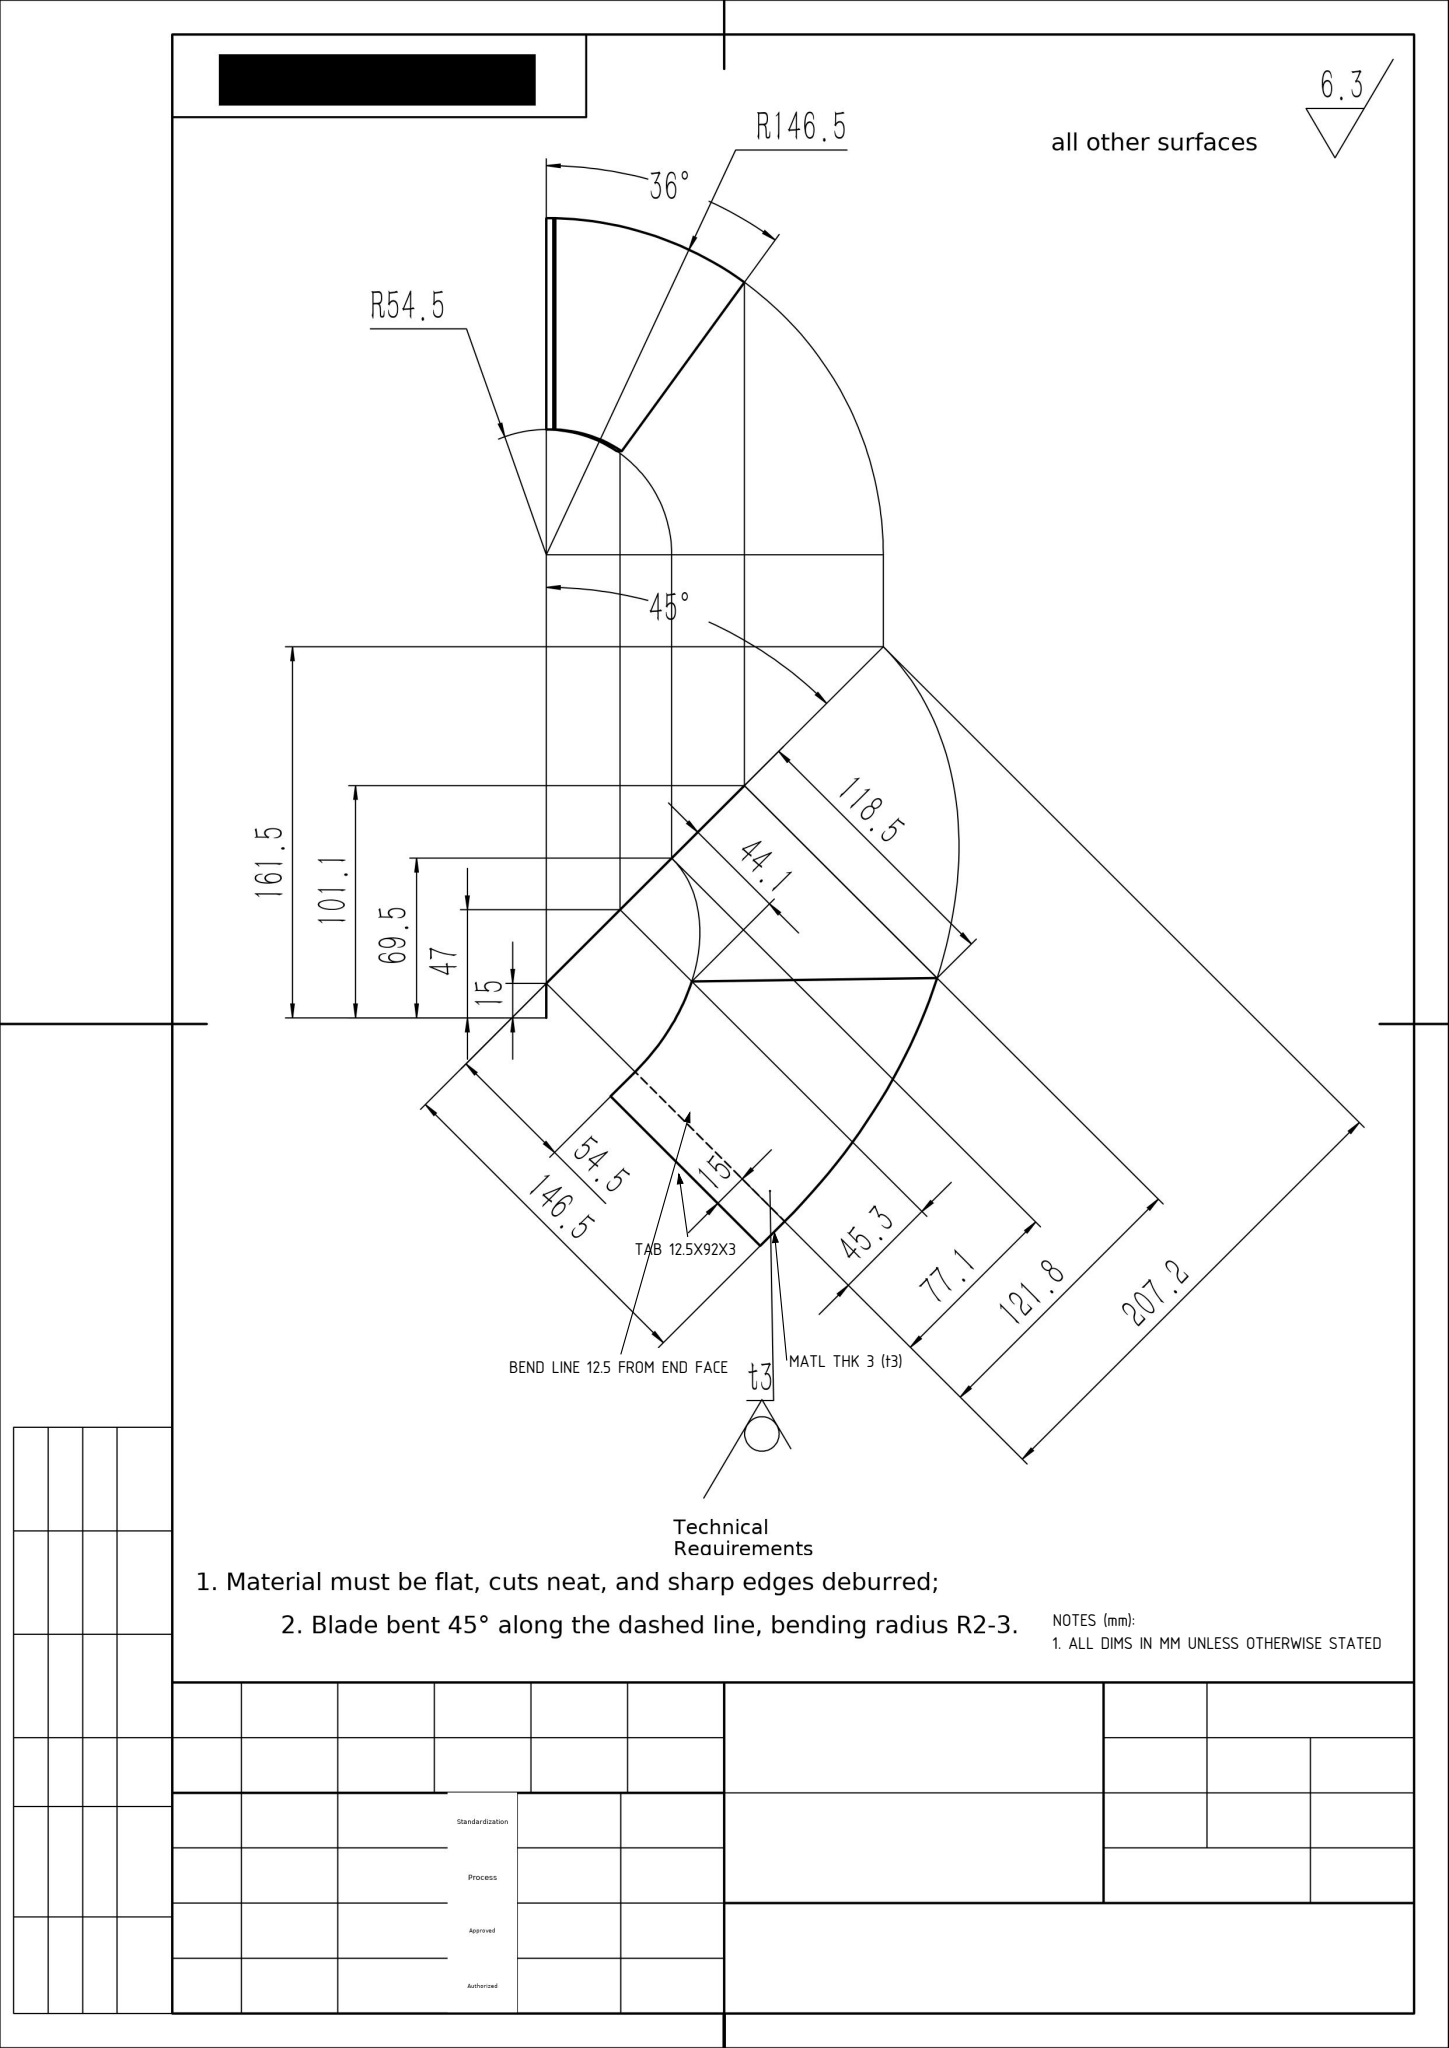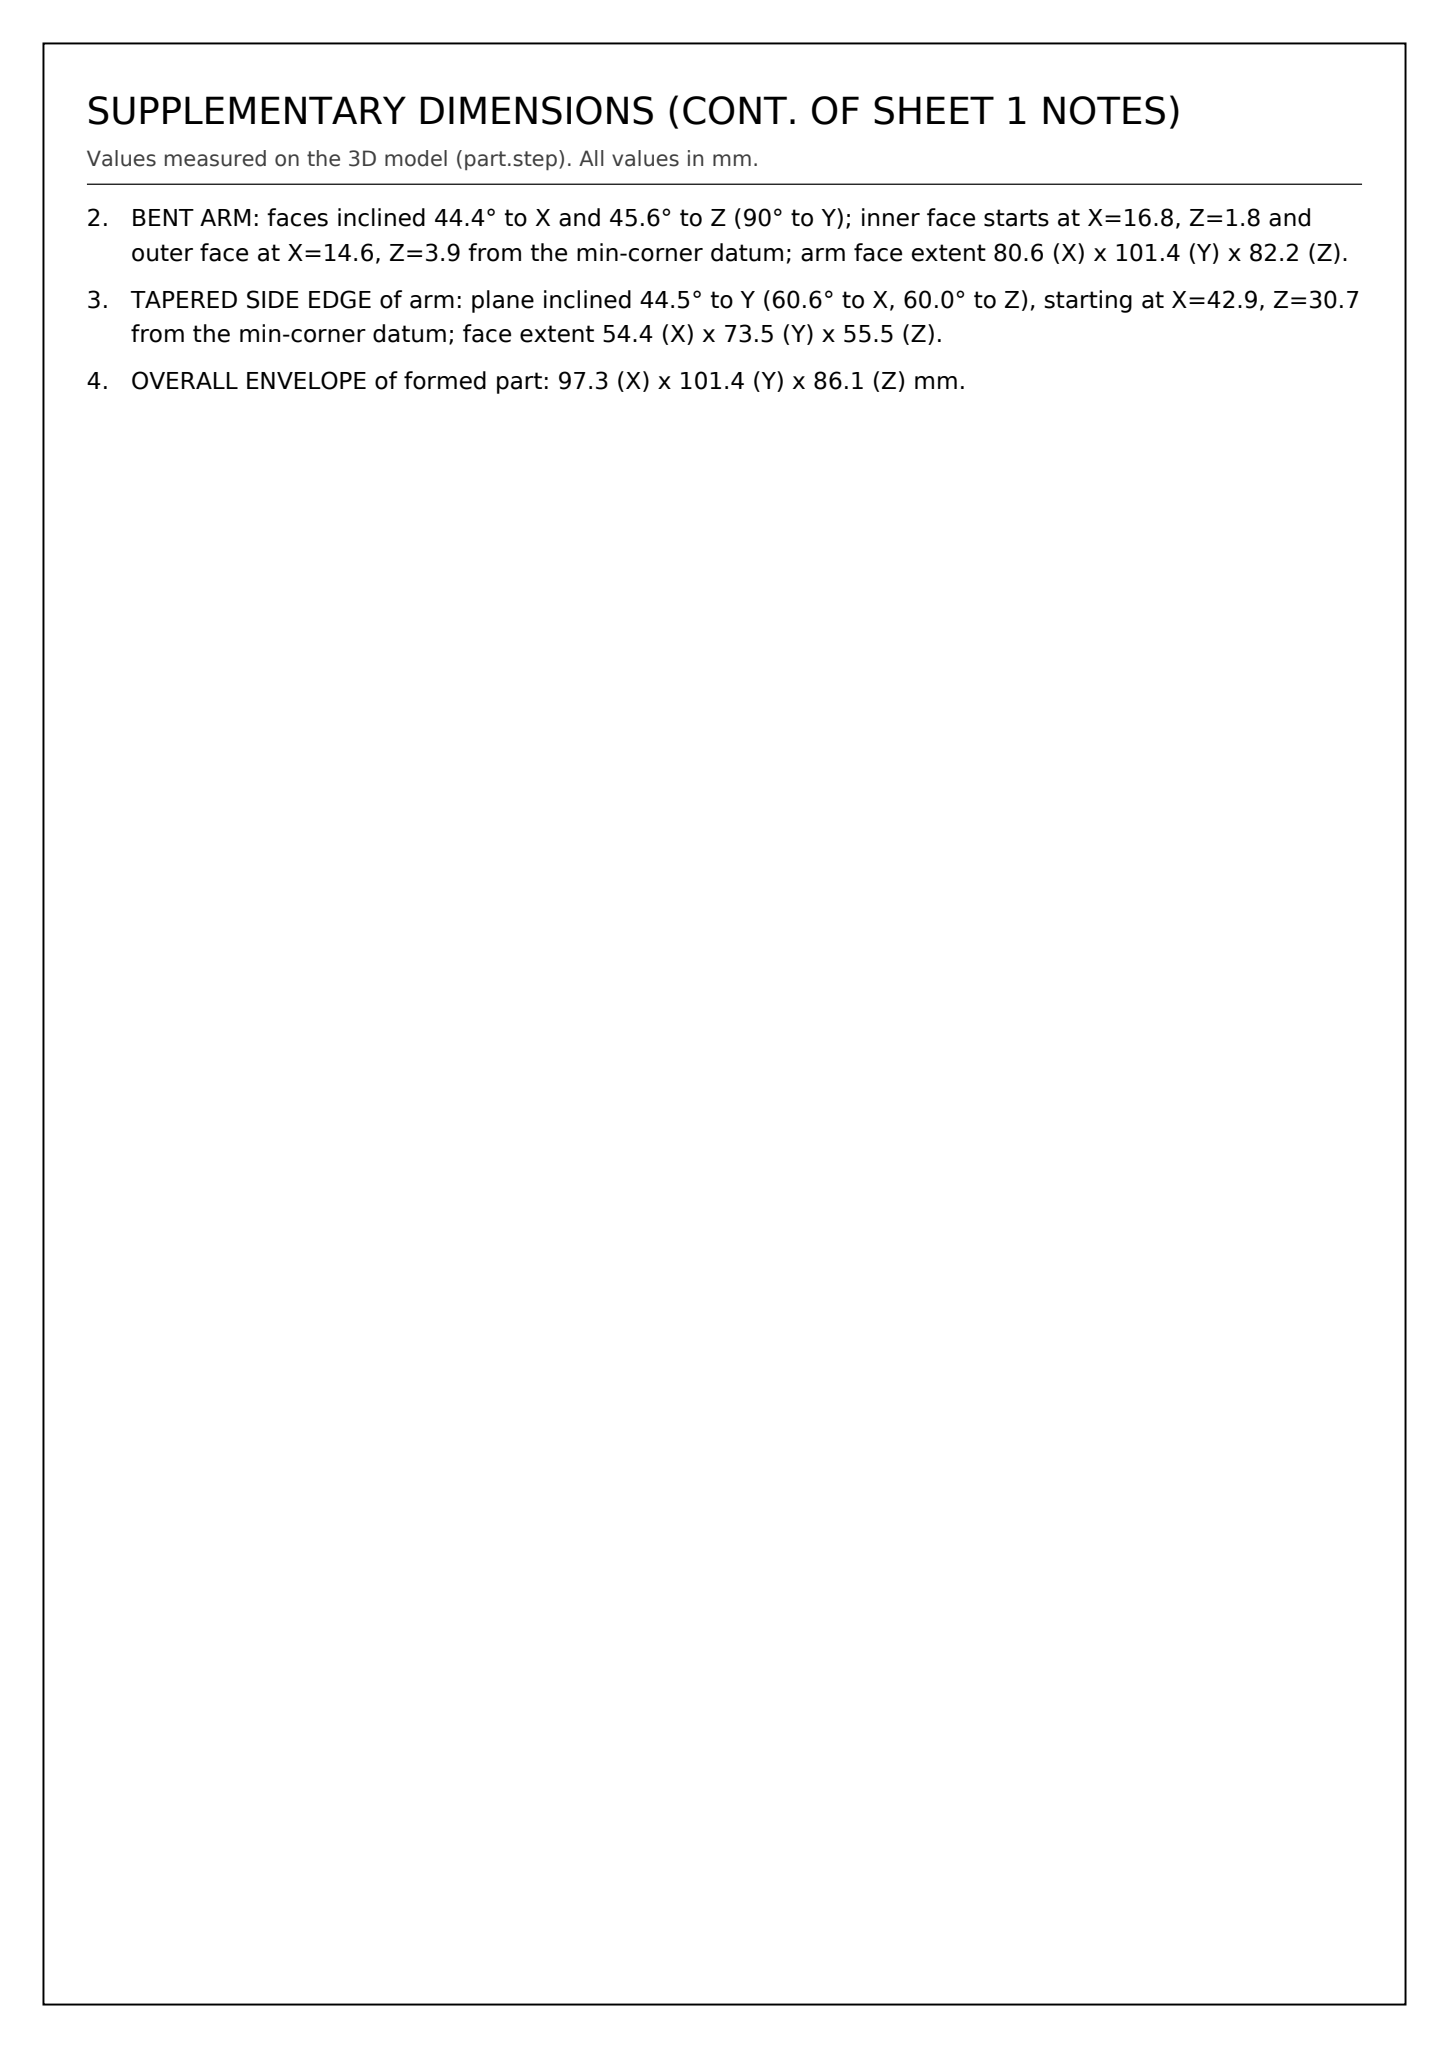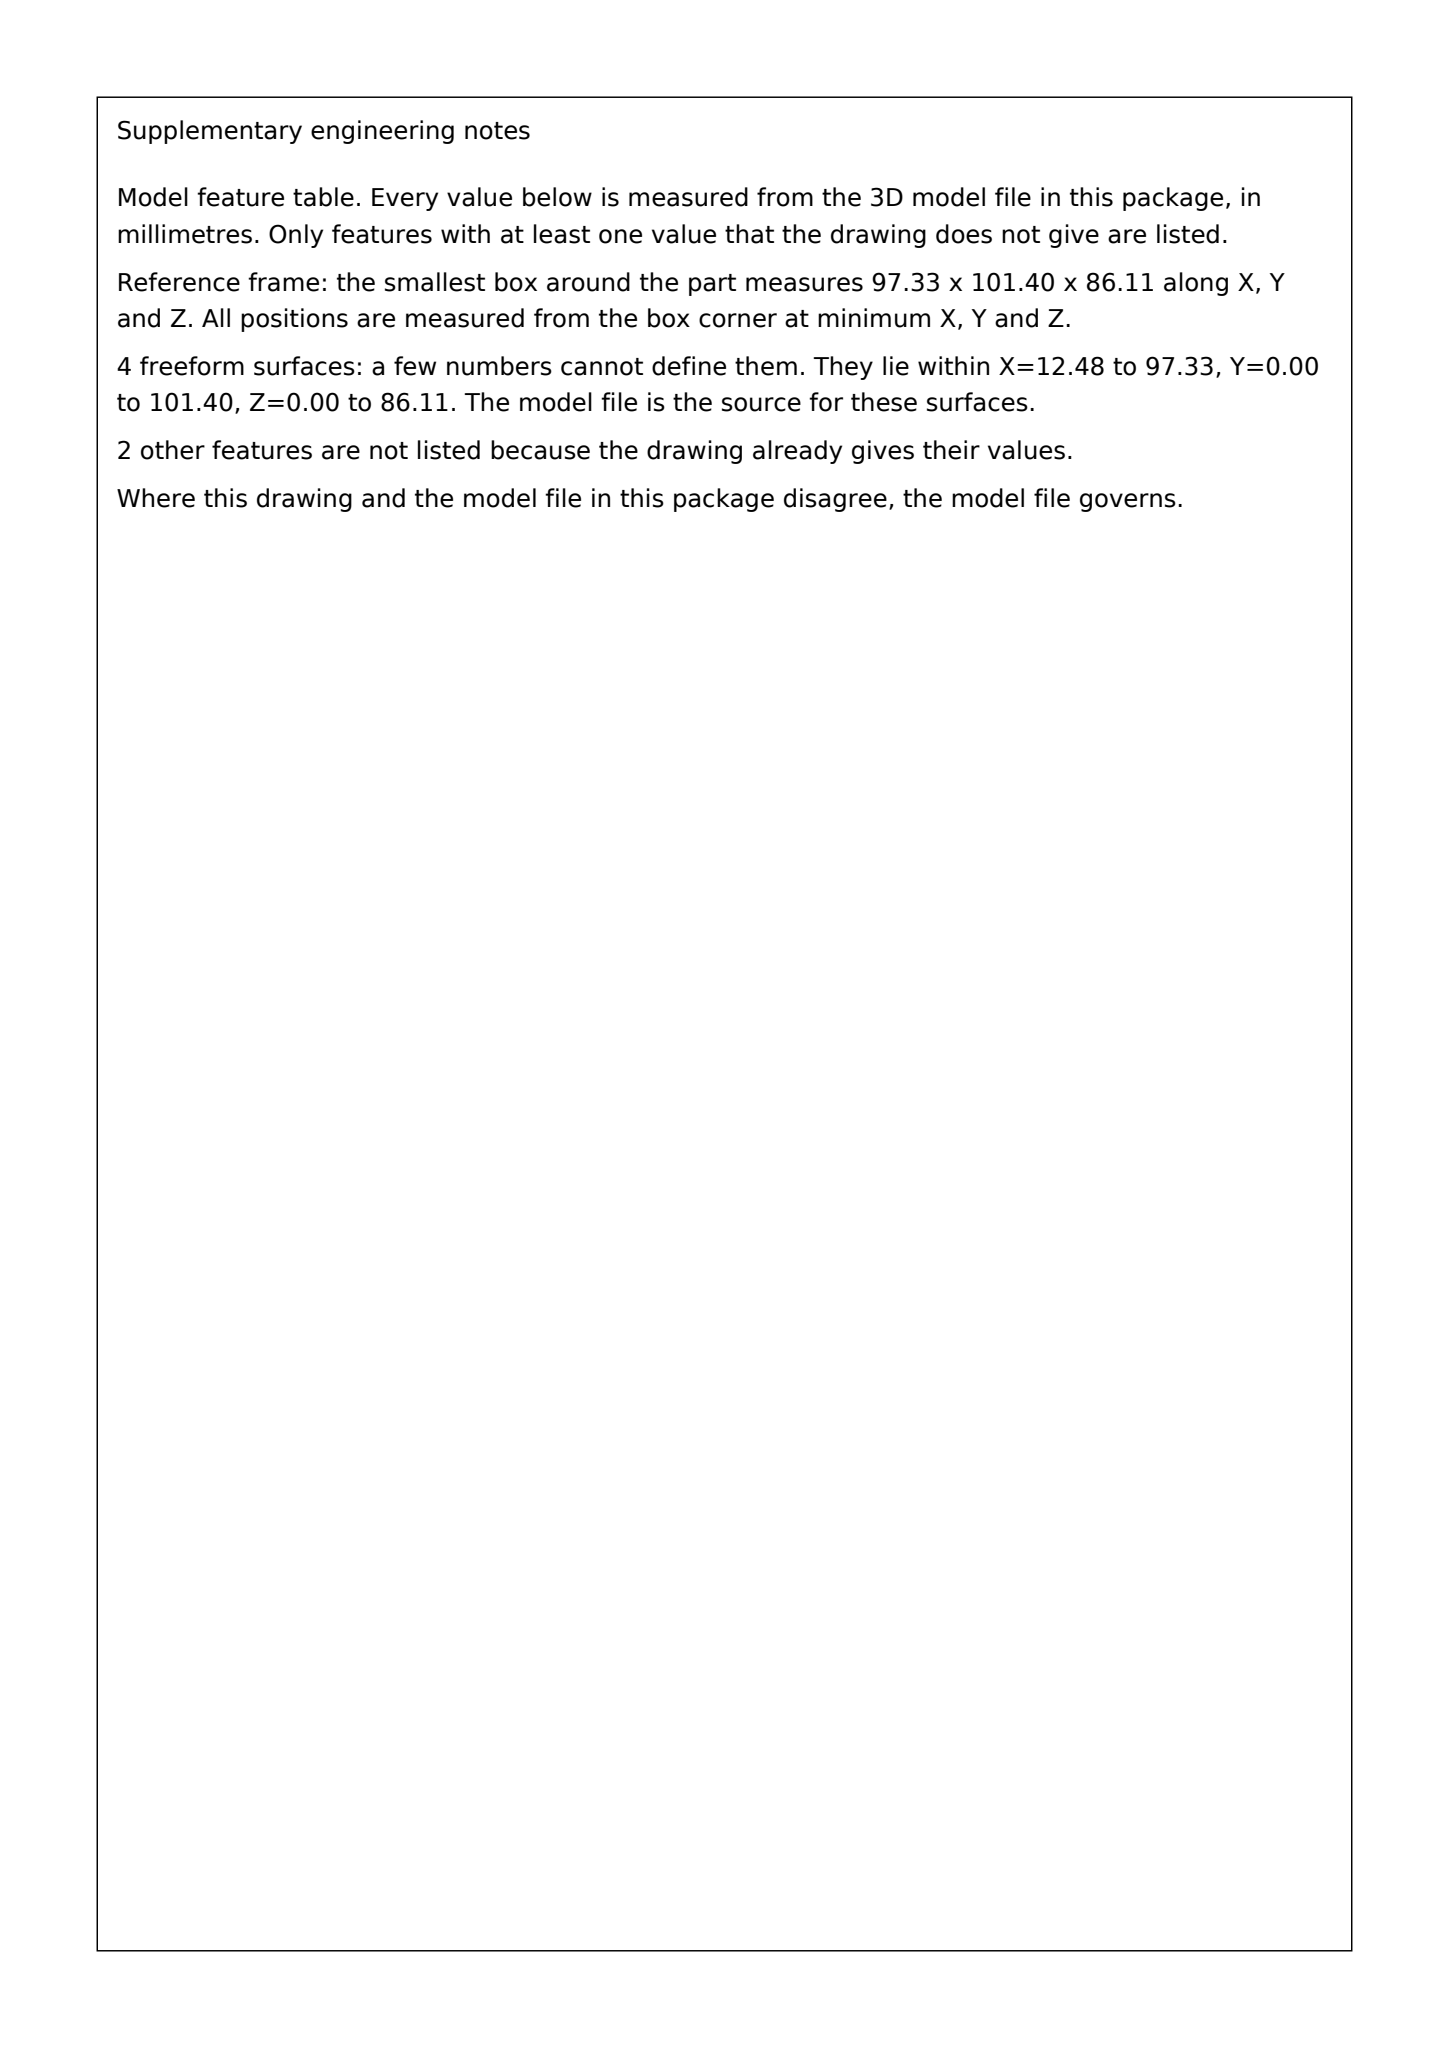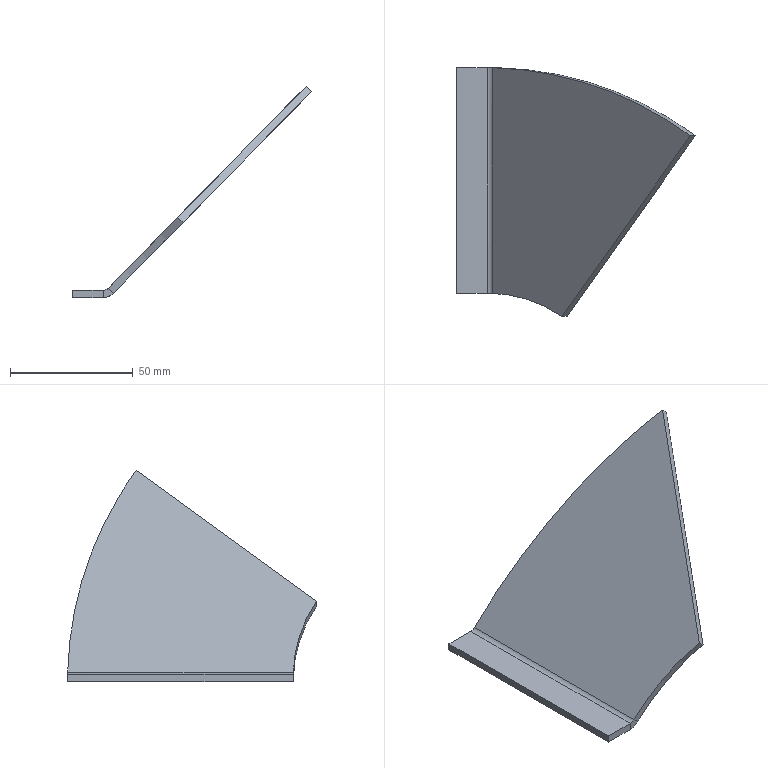Part | SolidWorks | mm | 1 solid | 14 faces | box 97.33 x 101.4 x 86.11 mm | volume 27238 mm3 | plane 8 | spline 4 | cylinder 2 | commonest cylinder face diameters 12 x1 6 x1
Drawing notes:
ALL DIMS IN MM UNLESS OTHERWISE STATED | from the solid: STEP model in mm: plate thk 3.00 (z 0.03 to 3.03) = drawing t3; bbox 97.331 x 101.401 x 86.141 consistent with 146.5/54.5 arc dims in mm
BENT ARM: faces inclined 44.4° to X and 45.6° to Z (90° to Y); inner face starts at X=16.8, Z=1.8 and outer face at X=14.6, Z=3.9 from the min-corner datum; arm face extent 80.6 (X) x 101.4 (Y) x 82.2 (Z). | from the solid: inclined_planes angle_to_xyz_axes [44.4,90.0,45.6], bbox_from [14.6,0.0,3.9] and [16.8,0.0,1.8], size [80.6,101.4,82.2]
TAPERED SIDE EDGE of arm: plane inclined 44.5° to Y (60.6° to X, 60.0° to Z), starting at X=42.9, Z=30.7 from the min-corner datum; face extent 54.4 (X) x 73.5 (Y) x 55.5 (Z). | from the solid: inclined_planes angle_to_xyz_axes [60.6,44.5,60.0], bbox_from [42.9,0.0,30.7], size [54.4,73.5,55.5]
OVERALL ENVELOPE of formed part: 97.3 (X) x 101.4 (Y) x 86.1 (Z) mm. | from the solid: bbox_xyz [97.331,101.401,86.141]
FLAT TAB 12.5X92X3: START 9.4 FROM END OF 101.4 EDGE | from the solid: Planes z=0/3 extent x[0,12.5] y[9.4,101.4]; bbox y=101.401
MATL THK 3 (t3) - RELOCATE CALLOUT CLEAR OF EXT LINES | from the solid: Tab faces z=0 and z=3, thickness 3
BEND LINE 12.5 FROM END FACE (DELETE 15) | from the solid: Tab x extent 0 to 12.5; arc axes at x=12.5
STEP:
#1=CARTESIAN_POINT('',(-147.378,146.448,3.9));
#2=VERTEX_POINT('',#1);
#3=CARTESIAN_POINT('',(-66.812,118.521,86.111));
#4=VERTEX_POINT('',#3);
#5=CARTESIAN_POINT('',(-147.378,146.448,3.9));
#6=CARTESIAN_POINT('',(-118.151,145.654,33.724));
#7=CARTESIAN_POINT('',(-90.466,136.057,61.974));
#8=CARTESIAN_POINT('',(-66.812,118.521,86.111));
#9=(BOUNDED_CURVE()B_SPLINE_CURVE(3,(#5,#6,#7,#8),.UNSPECIFIED.,.F.,.F.)B_SPLINE_CURVE_WITH_KNOTS((4,4),(4.739,5.341),.UNSPECIFIED.)CURVE()GEOMETRIC_REPRESENTATION_ITEM()RATIONAL_B_SPLINE_CURVE((1.,0.9701,0.9701,1.))REPRESENTATION_ITEM(''));
#10=EDGE_CURVE('',#2,#4,#9,.T.);
#11=ORIENTED_EDGE('',*,*,#10,.F.);
#12=CARTESIAN_POINT('',(-147.378,54.47,3.9));
#13=VERTEX_POINT('',#12);
#14=CARTESIAN_POINT('',(-147.378,147.,3.9));
#15=DIRECTION('',(0.,-1.,0.));
#16=VECTOR('',#15,1000.);
#17=LINE('',#14,#16);
#18=EDGE_CURVE('',#2,#13,#17,.T.);
#19=ORIENTED_EDGE('',*,*,#18,.T.);
#20=CARTESIAN_POINT('',(-119.111,45.069,32.744));
#21=VERTEX_POINT('',#20);
#22=CARTESIAN_POINT('',(-119.111,45.069,32.744));
#23=CARTESIAN_POINT('',(-127.528,50.908,24.155));
#24=CARTESIAN_POINT('',(-137.205,54.127,14.281));
#25=CARTESIAN_POINT('',(-147.378,54.47,3.9));
#26=(BOUNDED_CURVE()B_SPLINE_CURVE(3,(#22,#23,#24,#25),.UNSPECIFIED.,.F.,.F.)B_SPLINE_CURVE_WITH_KNOTS((4,4),(0.9737,1.538),.UNSPECIFIED.)CURVE()GEOMETRIC_REPRESENTATION_ITEM()RATIONAL_B_SPLINE_CURVE((1.,0.9737,0.9737,1.))REPRESENTATION_ITEM(''));
#27=EDGE_CURVE('',#21,#13,#26,.T.);
#28=ORIENTED_EDGE('',*,*,#27,.F.);
#29=CARTESIAN_POINT('',(-98.717,73.712,53.555));
#30=DIRECTION('',(-0.4991,-0.701,-0.5093));
#31=VECTOR('',#30,1000.);
#32=LINE('',#29,#31);
#33=EDGE_CURVE('',#4,#21,#32,.T.);
#34=ORIENTED_EDGE('',*,*,#33,.F.);
#35=EDGE_LOOP('',(#11,#19,#28,#34));
#36=FACE_OUTER_BOUND('',#35,.T.);
#37=CARTESIAN_POINT('',(-149.143,147.,2.1));
#38=DIRECTION('',(0.7142,0.,-0.6999));
#39=DIRECTION('',(-0.6999,0.,-0.7142));
#40=AXIS2_PLACEMENT_3D('',#37,#38,#39);
#41=PLANE('',#40);
#42=ADVANCED_FACE('',(#36),#41,.F.);
#43=CARTESIAN_POINT('',(-145.236,146.448,1.8));
#44=VERTEX_POINT('',#43);
#45=CARTESIAN_POINT('',(-145.236,54.47,1.8));
#46=VERTEX_POINT('',#45);
#47=CARTESIAN_POINT('',(-145.236,147.,1.8));
#48=DIRECTION('',(0.,-1.,0.));
#49=VECTOR('',#48,1000.);
#50=LINE('',#47,#49);
#51=EDGE_CURVE('',#44,#46,#50,.T.);
#52=ORIENTED_EDGE('',*,*,#51,.F.);
#53=CARTESIAN_POINT('',(-64.669,118.521,84.011));
#54=VERTEX_POINT('',#53);
#55=CARTESIAN_POINT('',(-145.236,146.448,1.8));
#56=CARTESIAN_POINT('',(-116.008,145.654,31.625));
#57=CARTESIAN_POINT('',(-88.324,136.057,59.874));
#58=CARTESIAN_POINT('',(-64.669,118.521,84.011));
#59=(BOUNDED_CURVE()B_SPLINE_CURVE(3,(#55,#56,#57,#58),.UNSPECIFIED.,.F.,.T.)B_SPLINE_CURVE_WITH_KNOTS((4,4),(4.739,5.341),.UNSPECIFIED.)CURVE()GEOMETRIC_REPRESENTATION_ITEM()RATIONAL_B_SPLINE_CURVE((1.,0.9701,0.9701,1.))REPRESENTATION_ITEM(''));
#60=EDGE_CURVE('',#44,#54,#59,.T.);
#61=ORIENTED_EDGE('',*,*,#60,.T.);
#62=CARTESIAN_POINT('',(-116.968,45.069,30.644));
#63=VERTEX_POINT('',#62);
#64=CARTESIAN_POINT('',(-96.574,73.712,51.455));
#65=DIRECTION('',(-0.4991,-0.701,-0.5093));
#66=VECTOR('',#65,1000.);
#67=LINE('',#64,#66);
#68=EDGE_CURVE('',#54,#63,#67,.T.);
#69=ORIENTED_EDGE('',*,*,#68,.T.);
#70=CARTESIAN_POINT('',(-116.968,45.069,30.644));
#71=CARTESIAN_POINT('',(-125.385,50.908,22.056));
#72=CARTESIAN_POINT('',(-135.063,54.127,12.181));
#73=CARTESIAN_POINT('',(-145.236,54.47,1.8));
#74=(BOUNDED_CURVE()B_SPLINE_CURVE(3,(#70,#71,#72,#73),.UNSPECIFIED.,.F.,.F.)B_SPLINE_CURVE_WITH_KNOTS((4,4),(0.9737,1.538),.UNSPECIFIED.)CURVE()GEOMETRIC_REPRESENTATION_ITEM()RATIONAL_B_SPLINE_CURVE((1.,0.9737,0.9737,1.))REPRESENTATION_ITEM(''));
#75=EDGE_CURVE('',#63,#46,#74,.T.);
#76=ORIENTED_EDGE('',*,*,#75,.T.);
#77=EDGE_LOOP('',(#52,#61,#69,#76));
#78=FACE_OUTER_BOUND('',#77,.T.);
#79=CARTESIAN_POINT('',(-147.,147.,0.));
#80=DIRECTION('',(0.7142,0.,-0.6999));
#81=DIRECTION('',(-0.6999,0.,-0.7142));
#82=AXIS2_PLACEMENT_3D('',#79,#80,#81);
#83=PLANE('',#82);
#84=ADVANCED_FACE('',(#78),#83,.T.);
#85=CARTESIAN_POINT('',(-149.521,146.469,0.));
#86=VERTEX_POINT('',#85);
#87=CARTESIAN_POINT('',(-149.521,54.5,0.));
#88=VERTEX_POINT('',#87);
#89=CARTESIAN_POINT('',(-149.521,147.,0.));
#90=DIRECTION('',(0.,-1.,0.));
#91=VECTOR('',#90,1000.);
#92=LINE('',#89,#91);
#93=EDGE_CURVE('',#86,#88,#92,.T.);
#94=ORIENTED_EDGE('',*,*,#93,.F.);
#95=CARTESIAN_POINT('',(-149.521,146.469,0.));
#96=CARTESIAN_POINT('',(-149.12,146.469,0.));
#97=CARTESIAN_POINT('',(-148.726,146.469,0.03981));
#98=CARTESIAN_POINT('',(-148.144,146.468,0.1568));
#99=CARTESIAN_POINT('',(-147.952,146.467,0.2054));
#100=CARTESIAN_POINT('',(-147.57,146.466,0.3224));
#101=CARTESIAN_POINT('',(-147.381,146.465,0.3909));
#102=CARTESIAN_POINT('',(-146.831,146.463,0.6219));
#103=CARTESIAN_POINT('',(-146.484,146.46,0.8103));
#104=CARTESIAN_POINT('',(-145.826,146.455,1.256));
#105=CARTESIAN_POINT('',(-145.516,146.452,1.514));
#106=CARTESIAN_POINT('',(-145.236,146.448,1.8));
#107=B_SPLINE_CURVE_WITH_KNOTS('',3,(#95,#96,#97,#98,#99,#100,#101,#102,#103,#104,#105,#106),.UNSPECIFIED.,.F.,.F.,(4,2,2,2,2,4),(0.,0.001186,0.001779,0.002372,0.003558,0.004744),.UNSPECIFIED.);
#108=EDGE_CURVE('',#86,#44,#107,.T.);
#109=ORIENTED_EDGE('',*,*,#108,.T.);
#110=ORIENTED_EDGE('',*,*,#51,.T.);
#111=CARTESIAN_POINT('',(-145.236,54.47,1.8));
#112=CARTESIAN_POINT('',(-145.516,54.48,1.514));
#113=CARTESIAN_POINT('',(-145.821,54.486,1.26));
#114=CARTESIAN_POINT('',(-146.311,54.492,0.9268));
#115=CARTESIAN_POINT('',(-146.481,54.494,0.8235));
#116=CARTESIAN_POINT('',(-146.831,54.496,0.6331));
#117=CARTESIAN_POINT('',(-147.012,54.497,0.546));
#118=CARTESIAN_POINT('',(-147.562,54.499,0.3148));
#119=CARTESIAN_POINT('',(-147.94,54.5,0.1984));
#120=CARTESIAN_POINT('',(-148.718,54.5,0.04068));
#121=CARTESIAN_POINT('',(-149.12,54.5,0.));
#122=CARTESIAN_POINT('',(-149.521,54.5,0.));
#123=B_SPLINE_CURVE_WITH_KNOTS('',3,(#111,#112,#113,#114,#115,#116,#117,#118,#119,#120,#121,#122),.UNSPECIFIED.,.F.,.F.,(4,2,2,2,2,4),(0.,0.001186,0.001779,0.002372,0.003558,0.004745),.UNSPECIFIED.);
#124=EDGE_CURVE('',#46,#88,#123,.T.);
#125=ORIENTED_EDGE('',*,*,#124,.T.);
#126=EDGE_LOOP('',(#94,#109,#110,#125));
#127=FACE_OUTER_BOUND('',#126,.T.);
#128=CARTESIAN_POINT('',(-149.521,147.,6.));
#129=DIRECTION('',(0.,-1.,0.));
#130=DIRECTION('',(0.,0.,-1.));
#131=AXIS2_PLACEMENT_3D('',#128,#129,#130);
#132=CYLINDRICAL_SURFACE('',#131,6.);
#133=ADVANCED_FACE('',(#127),#132,.T.);
#134=CARTESIAN_POINT('',(-162.,146.469,0.));
#135=VERTEX_POINT('',#134);
#136=CARTESIAN_POINT('',(-162.,54.5,0.));
#137=VERTEX_POINT('',#136);
#138=CARTESIAN_POINT('',(-162.,147.,0.));
#139=DIRECTION('',(0.,-1.,0.));
#140=VECTOR('',#139,1000.);
#141=LINE('',#138,#140);
#142=EDGE_CURVE('',#135,#137,#141,.T.);
#143=ORIENTED_EDGE('',*,*,#142,.F.);
#144=CARTESIAN_POINT('',(-162.,146.469,0.));
#145=DIRECTION('',(1.,0.,0.));
#146=VECTOR('',#145,1000.);
#147=LINE('',#144,#146);
#148=EDGE_CURVE('',#135,#86,#147,.T.);
#149=ORIENTED_EDGE('',*,*,#148,.T.);
#150=ORIENTED_EDGE('',*,*,#93,.T.);
#151=CARTESIAN_POINT('',(-162.,54.5,0.));
#152=DIRECTION('',(1.,0.,0.));
#153=VECTOR('',#152,1000.);
#154=LINE('',#151,#153);
#155=EDGE_CURVE('',#137,#88,#154,.T.);
#156=ORIENTED_EDGE('',*,*,#155,.F.);
#157=EDGE_LOOP('',(#143,#149,#150,#156));
#158=FACE_OUTER_BOUND('',#157,.T.);
#159=CARTESIAN_POINT('',(-162.,147.,0.));
#160=DIRECTION('',(0.,0.,-1.));
#161=DIRECTION('',(-1.,0.,-0.));
#162=AXIS2_PLACEMENT_3D('',#159,#160,#161);
#163=PLANE('',#162);
#164=ADVANCED_FACE('',(#158),#163,.T.);
#165=CARTESIAN_POINT('',(-162.,146.469,3.));
#166=VERTEX_POINT('',#165);
#167=CARTESIAN_POINT('',(-162.,54.5,3.));
#168=VERTEX_POINT('',#167);
#169=CARTESIAN_POINT('',(-162.,147.,3.));
#170=DIRECTION('',(0.,-1.,0.));
#171=VECTOR('',#170,1000.);
#172=LINE('',#169,#171);
#173=EDGE_CURVE('',#166,#168,#172,.T.);
#174=ORIENTED_EDGE('',*,*,#173,.F.);
#175=CARTESIAN_POINT('',(-162.,146.469,3.));
#176=DIRECTION('',(0.,0.,-1.));
#177=VECTOR('',#176,1000.);
#178=LINE('',#175,#177);
#179=EDGE_CURVE('',#166,#135,#178,.T.);
#180=ORIENTED_EDGE('',*,*,#179,.T.);
#181=ORIENTED_EDGE('',*,*,#142,.T.);
#182=CARTESIAN_POINT('',(-162.,54.5,0.));
#183=DIRECTION('',(-0.,0.,1.));
#184=VECTOR('',#183,1000.);
#185=LINE('',#182,#184);
#186=EDGE_CURVE('',#137,#168,#185,.T.);
#187=ORIENTED_EDGE('',*,*,#186,.T.);
#188=EDGE_LOOP('',(#174,#180,#181,#187));
#189=FACE_OUTER_BOUND('',#188,.T.);
#190=CARTESIAN_POINT('',(-162.,147.,3.));
#191=DIRECTION('',(-1.,0.,0.));
#192=DIRECTION('',(0.,0.,1.));
#193=AXIS2_PLACEMENT_3D('',#190,#191,#192);
#194=PLANE('',#193);
#195=ADVANCED_FACE('',(#189),#194,.T.);
#196=CARTESIAN_POINT('',(-149.521,146.469,3.));
#197=VERTEX_POINT('',#196);
#198=CARTESIAN_POINT('',(-162.,146.469,3.));
#199=DIRECTION('',(1.,0.,0.));
#200=VECTOR('',#199,1000.);
#201=LINE('',#198,#200);
#202=EDGE_CURVE('',#166,#197,#201,.T.);
#203=ORIENTED_EDGE('',*,*,#202,.F.);
#204=ORIENTED_EDGE('',*,*,#173,.T.);
#205=CARTESIAN_POINT('',(-149.521,54.5,3.));
#206=VERTEX_POINT('',#205);
#207=CARTESIAN_POINT('',(-162.,54.5,3.));
#208=DIRECTION('',(1.,0.,0.));
#209=VECTOR('',#208,1000.);
#210=LINE('',#207,#209);
#211=EDGE_CURVE('',#168,#206,#210,.T.);
#212=ORIENTED_EDGE('',*,*,#211,.T.);
#213=CARTESIAN_POINT('',(-149.521,147.,3.));
#214=DIRECTION('',(0.,-1.,0.));
#215=VECTOR('',#214,1000.);
#216=LINE('',#213,#215);
#217=EDGE_CURVE('',#197,#206,#216,.T.);
#218=ORIENTED_EDGE('',*,*,#217,.F.);
#219=EDGE_LOOP('',(#203,#204,#212,#218));
#220=FACE_OUTER_BOUND('',#219,.T.);
#221=CARTESIAN_POINT('',(-162.,147.,3.));
#222=DIRECTION('',(0.,0.,-1.));
#223=DIRECTION('',(-1.,0.,-0.));
#224=AXIS2_PLACEMENT_3D('',#221,#222,#223);
#225=PLANE('',#224);
#226=ADVANCED_FACE('',(#220),#225,.F.);
#227=CARTESIAN_POINT('',(-149.521,146.469,3.));
#228=CARTESIAN_POINT('',(-149.321,146.469,3.));
#229=CARTESIAN_POINT('',(-149.123,146.469,3.02));
#230=CARTESIAN_POINT('',(-148.733,146.467,3.099));
#231=CARTESIAN_POINT('',(-148.541,146.466,3.158));
#232=CARTESIAN_POINT('',(-147.995,146.461,3.387));
#233=CARTESIAN_POINT('',(-147.658,146.456,3.614));
#234=CARTESIAN_POINT('',(-147.378,146.448,3.9));
#235=B_SPLINE_CURVE_WITH_KNOTS('',3,(#227,#228,#229,#230,#231,#232,#233,#234),.UNSPECIFIED.,.F.,.F.,(4,2,2,4),(0.,0.0005959,0.001192,0.002383),.UNSPECIFIED.);
#236=EDGE_CURVE('',#197,#2,#235,.T.);
#237=ORIENTED_EDGE('',*,*,#236,.F.);
#238=ORIENTED_EDGE('',*,*,#217,.T.);
#239=CARTESIAN_POINT('',(-147.378,54.47,3.9));
#240=CARTESIAN_POINT('',(-147.518,54.48,3.757));
#241=CARTESIAN_POINT('',(-147.671,54.486,3.63));
#242=CARTESIAN_POINT('',(-148.,54.494,3.406));
#243=CARTESIAN_POINT('',(-148.177,54.497,3.311));
#244=CARTESIAN_POINT('',(-148.723,54.501,3.081));
#245=CARTESIAN_POINT('',(-149.12,54.5,3.));
#246=CARTESIAN_POINT('',(-149.521,54.5,3.));
#247=B_SPLINE_CURVE_WITH_KNOTS('',3,(#239,#240,#241,#242,#243,#244,#245,#246),.UNSPECIFIED.,.F.,.F.,(4,2,2,4),(0.,0.0005959,0.001192,0.002384),.UNSPECIFIED.);
#248=EDGE_CURVE('',#13,#206,#247,.T.);
#249=ORIENTED_EDGE('',*,*,#248,.F.);
#250=ORIENTED_EDGE('',*,*,#18,.F.);
#251=EDGE_LOOP('',(#237,#238,#249,#250));
#252=FACE_OUTER_BOUND('',#251,.T.);
#253=CARTESIAN_POINT('',(-149.521,147.,6.));
#254=DIRECTION('',(0.,-1.,0.));
#255=DIRECTION('',(0.,0.,-1.));
#256=AXIS2_PLACEMENT_3D('',#253,#254,#255);
#257=CYLINDRICAL_SURFACE('',#256,3.);
#258=ADVANCED_FACE('',(#252),#257,.F.);
#259=CARTESIAN_POINT('',(-116.968,45.069,30.644));
#260=DIRECTION('',(0.7142,0.,-0.6999));
#261=VECTOR('',#260,1000.);
#262=LINE('',#259,#261);
#263=EDGE_CURVE('',#21,#63,#262,.T.);
#264=ORIENTED_EDGE('',*,*,#263,.T.);
#265=ORIENTED_EDGE('',*,*,#68,.F.);
#266=CARTESIAN_POINT('',(-66.812,118.521,86.111));
#267=DIRECTION('',(0.7142,0.,-0.6999));
#268=VECTOR('',#267,1000.);
#269=LINE('',#266,#268);
#270=EDGE_CURVE('',#4,#54,#269,.T.);
#271=ORIENTED_EDGE('',*,*,#270,.F.);
#272=ORIENTED_EDGE('',*,*,#33,.T.);
#273=EDGE_LOOP('',(#264,#265,#271,#272));
#274=FACE_OUTER_BOUND('',#273,.T.);
#275=CARTESIAN_POINT('',(-98.717,73.712,53.555));
#276=DIRECTION('',(0.4907,-0.7131,0.5007));
#277=DIRECTION('',(-0.4991,-0.701,-0.5093));
#278=AXIS2_PLACEMENT_3D('',#275,#276,#277);
#279=PLANE('',#278);
#280=ADVANCED_FACE('',(#274),#279,.T.);
#281=ORIENTED_EDGE('',*,*,#10,.T.);
#282=ORIENTED_EDGE('',*,*,#270,.T.);
#283=ORIENTED_EDGE('',*,*,#60,.F.);
#284=CARTESIAN_POINT('',(-147.378,146.448,3.9));
#285=DIRECTION('',(0.7142,0.,-0.6999));
#286=VECTOR('',#285,1000.);
#287=LINE('',#284,#286);
#288=EDGE_CURVE('',#2,#44,#287,.T.);
#289=ORIENTED_EDGE('',*,*,#288,.F.);
#290=EDGE_LOOP('',(#281,#282,#283,#289));
#291=FACE_OUTER_BOUND('',#290,.T.);
#292=CARTESIAN_POINT('',(-147.378,146.448,3.9));
#293=CARTESIAN_POINT('',(-145.236,146.448,1.8));
#294=CARTESIAN_POINT('',(-118.151,145.654,33.724));
#295=CARTESIAN_POINT('',(-116.008,145.654,31.625));
#296=CARTESIAN_POINT('',(-90.466,136.057,61.974));
#297=CARTESIAN_POINT('',(-88.324,136.057,59.874));
#298=CARTESIAN_POINT('',(-66.812,118.521,86.111));
#299=CARTESIAN_POINT('',(-64.669,118.521,84.011));
#300=(BOUNDED_SURFACE()B_SPLINE_SURFACE(3,1,((#292,#293),(#294,#295),(#296,#297),(#298,#299)),.UNSPECIFIED.,.F.,.F.,.F.)B_SPLINE_SURFACE_WITH_KNOTS((4,4),(2,2),(0.,1.),(0.,1.),.UNSPECIFIED.)GEOMETRIC_REPRESENTATION_ITEM()RATIONAL_B_SPLINE_SURFACE(((1.,1.),(0.9701,0.9701),(0.9701,0.9701),(1.,1.)))REPRESENTATION_ITEM('')SURFACE());
#301=ADVANCED_FACE('',(#291),#300,.T.);
#302=ORIENTED_EDGE('',*,*,#27,.T.);
#303=CARTESIAN_POINT('',(-145.236,54.47,1.8));
#304=DIRECTION('',(-0.7142,0.,0.6999));
#305=VECTOR('',#304,1000.);
#306=LINE('',#303,#305);
#307=EDGE_CURVE('',#46,#13,#306,.T.);
#308=ORIENTED_EDGE('',*,*,#307,.F.);
#309=ORIENTED_EDGE('',*,*,#75,.F.);
#310=ORIENTED_EDGE('',*,*,#263,.F.);
#311=EDGE_LOOP('',(#302,#308,#309,#310));
#312=FACE_OUTER_BOUND('',#311,.T.);
#313=CARTESIAN_POINT('',(-119.111,45.069,32.744));
#314=CARTESIAN_POINT('',(-116.968,45.069,30.644));
#315=CARTESIAN_POINT('',(-127.528,50.908,24.155));
#316=CARTESIAN_POINT('',(-125.385,50.908,22.056));
#317=CARTESIAN_POINT('',(-137.205,54.127,14.281));
#318=CARTESIAN_POINT('',(-135.063,54.127,12.181));
#319=CARTESIAN_POINT('',(-147.378,54.47,3.9));
#320=CARTESIAN_POINT('',(-145.236,54.47,1.8));
#321=(BOUNDED_SURFACE()B_SPLINE_SURFACE(3,1,((#313,#314),(#315,#316),(#317,#318),(#319,#320)),.UNSPECIFIED.,.F.,.F.,.T.)B_SPLINE_SURFACE_WITH_KNOTS((4,4),(2,2),(0.,1.),(0.,1.),.UNSPECIFIED.)GEOMETRIC_REPRESENTATION_ITEM()RATIONAL_B_SPLINE_SURFACE(((1.,1.),(0.9737,0.9737),(0.9737,0.9737),(1.,1.)))REPRESENTATION_ITEM('')SURFACE());
#322=ADVANCED_FACE('',(#312),#321,.F.);
#323=ORIENTED_EDGE('',*,*,#202,.T.);
#324=CARTESIAN_POINT('',(-149.521,146.469,3.));
#325=DIRECTION('',(0.,0.,-1.));
#326=VECTOR('',#325,1000.);
#327=LINE('',#324,#326);
#328=EDGE_CURVE('',#197,#86,#327,.T.);
#329=ORIENTED_EDGE('',*,*,#328,.T.);
#330=ORIENTED_EDGE('',*,*,#148,.F.);
#331=ORIENTED_EDGE('',*,*,#179,.F.);
#332=EDGE_LOOP('',(#323,#329,#330,#331));
#333=FACE_OUTER_BOUND('',#332,.T.);
#334=CARTESIAN_POINT('',(-162.,146.469,3.));
#335=DIRECTION('',(0.,1.,0.));
#336=DIRECTION('',(1.,0.,0.));
#337=AXIS2_PLACEMENT_3D('',#334,#335,#336);
#338=PLANE('',#337);
#339=ADVANCED_FACE('',(#333),#338,.T.);
#340=ORIENTED_EDGE('',*,*,#236,.T.);
#341=ORIENTED_EDGE('',*,*,#288,.T.);
#342=ORIENTED_EDGE('',*,*,#108,.F.);
#343=ORIENTED_EDGE('',*,*,#328,.F.);
#344=EDGE_LOOP('',(#340,#341,#342,#343));
#345=FACE_OUTER_BOUND('',#344,.T.);
#346=CARTESIAN_POINT('',(-149.521,146.469,3.03));
#347=CARTESIAN_POINT('',(-149.322,146.469,3.03));
#348=CARTESIAN_POINT('',(-149.127,146.469,3.05));
#349=CARTESIAN_POINT('',(-148.839,146.468,3.108));
#350=CARTESIAN_POINT('',(-148.744,146.467,3.132));
#351=CARTESIAN_POINT('',(-148.555,146.466,3.19));
#352=CARTESIAN_POINT('',(-148.462,146.465,3.224));
#353=CARTESIAN_POINT('',(-148.19,146.463,3.338));
#354=CARTESIAN_POINT('',(-148.018,146.46,3.431));
#355=CARTESIAN_POINT('',(-147.692,146.455,3.652));
#356=CARTESIAN_POINT('',(-147.538,146.452,3.78));
#357=CARTESIAN_POINT('',(-147.4,146.448,3.921));
#358=CARTESIAN_POINT('',(-149.521,146.469,3.));
#359=CARTESIAN_POINT('',(-149.32,146.469,3.));
#360=CARTESIAN_POINT('',(-149.123,146.469,3.02));
#361=CARTESIAN_POINT('',(-148.832,146.468,3.078));
#362=CARTESIAN_POINT('',(-148.736,146.467,3.103));
#363=CARTESIAN_POINT('',(-148.546,146.466,3.161));
#364=CARTESIAN_POINT('',(-148.451,146.465,3.195));
#365=CARTESIAN_POINT('',(-148.176,146.463,3.311));
#366=CARTESIAN_POINT('',(-148.002,146.46,3.405));
#367=CARTESIAN_POINT('',(-147.674,146.455,3.628));
#368=CARTESIAN_POINT('',(-147.518,146.452,3.757));
#369=CARTESIAN_POINT('',(-147.378,146.448,3.9));
#370=CARTESIAN_POINT('',(-149.521,146.469,0.));
#371=CARTESIAN_POINT('',(-149.12,146.469,0.));
#372=CARTESIAN_POINT('',(-148.725,146.469,0.03981));
#373=CARTESIAN_POINT('',(-148.144,146.468,0.1568));
#374=CARTESIAN_POINT('',(-147.952,146.467,0.2054));
#375=CARTESIAN_POINT('',(-147.57,146.466,0.3224));
#376=CARTESIAN_POINT('',(-147.381,146.465,0.391));
#377=CARTESIAN_POINT('',(-146.831,146.463,0.6219));
#378=CARTESIAN_POINT('',(-146.484,146.46,0.8104));
#379=CARTESIAN_POINT('',(-145.826,146.455,1.256));
#380=CARTESIAN_POINT('',(-145.516,146.452,1.515));
#381=CARTESIAN_POINT('',(-145.236,146.448,1.8));
#382=CARTESIAN_POINT('',(-149.521,146.469,-0.03));
#383=CARTESIAN_POINT('',(-149.118,146.469,-0.03));
#384=CARTESIAN_POINT('',(-148.721,146.469,0.01001));
#385=CARTESIAN_POINT('',(-148.137,146.468,0.1276));
#386=CARTESIAN_POINT('',(-147.944,146.467,0.1765));
#387=CARTESIAN_POINT('',(-147.561,146.466,0.294));
#388=CARTESIAN_POINT('',(-147.37,146.465,0.3629));
#389=CARTESIAN_POINT('',(-146.818,146.463,0.5951));
#390=CARTESIAN_POINT('',(-146.468,146.46,0.7844));
#391=CARTESIAN_POINT('',(-145.808,146.455,1.232));
#392=CARTESIAN_POINT('',(-145.496,146.452,1.492));
#393=CARTESIAN_POINT('',(-145.214,146.448,1.779));
#394=B_SPLINE_SURFACE_WITH_KNOTS('',1,3,((#346,#347,#348,#349,#350,#351,#352,#353,#354,#355,#356,#357),(#358,#359,#360,#361,#362,#363,#364,#365,#366,#367,#368,#369),(#370,#371,#372,#373,#374,#375,#376,#377,#378,#379,#380,#381),(#382,#383,#384,#385,#386,#387,#388,#389,#390,#391,#392,#393)),.UNSPECIFIED.,.F.,.F.,.F.,(2,1,1,2),(4,2,2,2,2,4),(-0.0101,0.,1.,1.01),(0.,0.0005931,0.0008896,0.001186,0.001779,0.002372),.UNSPECIFIED.);
#395=ADVANCED_FACE('',(#345),#394,.F.);
#396=ORIENTED_EDGE('',*,*,#186,.F.);
#397=ORIENTED_EDGE('',*,*,#155,.T.);
#398=CARTESIAN_POINT('',(-149.521,54.5,0.));
#399=DIRECTION('',(-0.,0.,1.));
#400=VECTOR('',#399,1000.);
#401=LINE('',#398,#400);
#402=EDGE_CURVE('',#88,#206,#401,.T.);
#403=ORIENTED_EDGE('',*,*,#402,.T.);
#404=ORIENTED_EDGE('',*,*,#211,.F.);
#405=EDGE_LOOP('',(#396,#397,#403,#404));
#406=FACE_OUTER_BOUND('',#405,.T.);
#407=CARTESIAN_POINT('',(-162.,54.5,0.));
#408=DIRECTION('',(0.,1.,0.));
#409=DIRECTION('',(1.,0.,0.));
#410=AXIS2_PLACEMENT_3D('',#407,#408,#409);
#411=PLANE('',#410);
#412=ADVANCED_FACE('',(#406),#411,.F.);
#413=ORIENTED_EDGE('',*,*,#402,.F.);
#414=ORIENTED_EDGE('',*,*,#124,.F.);
#415=ORIENTED_EDGE('',*,*,#307,.T.);
#416=ORIENTED_EDGE('',*,*,#248,.T.);
#417=EDGE_LOOP('',(#413,#414,#415,#416));
#418=FACE_OUTER_BOUND('',#417,.T.);
#419=CARTESIAN_POINT('',(-147.4,54.47,3.921));
#420=CARTESIAN_POINT('',(-147.539,54.48,3.779));
#421=CARTESIAN_POINT('',(-147.689,54.486,3.654));
#422=CARTESIAN_POINT('',(-148.013,54.494,3.434));
#423=CARTESIAN_POINT('',(-148.188,54.497,3.338));
#424=CARTESIAN_POINT('',(-148.733,54.501,3.11));
#425=CARTESIAN_POINT('',(-149.121,54.5,3.03));
#426=CARTESIAN_POINT('',(-149.521,54.5,3.03));
#427=CARTESIAN_POINT('',(-147.378,54.47,3.9));
#428=CARTESIAN_POINT('',(-147.519,54.48,3.757));
#429=CARTESIAN_POINT('',(-147.671,54.486,3.63));
#430=CARTESIAN_POINT('',(-147.998,54.494,3.408));
#431=CARTESIAN_POINT('',(-148.175,54.497,3.312));
#432=CARTESIAN_POINT('',(-148.725,54.501,3.08));
#433=CARTESIAN_POINT('',(-149.117,54.5,3.));
#434=CARTESIAN_POINT('',(-149.521,54.5,3.));
#435=CARTESIAN_POINT('',(-145.236,54.47,1.8));
#436=CARTESIAN_POINT('',(-145.516,54.48,1.514));
#437=CARTESIAN_POINT('',(-145.821,54.486,1.26));
#438=CARTESIAN_POINT('',(-146.475,54.494,0.8156));
#439=CARTESIAN_POINT('',(-146.829,54.497,0.623));
#440=CARTESIAN_POINT('',(-147.929,54.501,0.1606));
#441=CARTESIAN_POINT('',(-148.713,54.5,0.));
#442=CARTESIAN_POINT('',(-149.521,54.5,0.));
#443=CARTESIAN_POINT('',(-145.214,54.47,1.779));
#444=CARTESIAN_POINT('',(-145.496,54.48,1.491));
#445=CARTESIAN_POINT('',(-145.802,54.486,1.236));
#446=CARTESIAN_POINT('',(-146.459,54.494,0.7894));
#447=CARTESIAN_POINT('',(-146.815,54.497,0.5959));
#448=CARTESIAN_POINT('',(-147.921,54.501,0.1311));
#449=CARTESIAN_POINT('',(-148.709,54.5,-0.0303));
#450=CARTESIAN_POINT('',(-149.521,54.5,-0.0303));
#451=B_SPLINE_SURFACE_WITH_KNOTS('',1,3,((#419,#420,#421,#422,#423,#424,#425,#426),(#427,#428,#429,#430,#431,#432,#433,#434),(#435,#436,#437,#438,#439,#440,#441,#442),(#443,#444,#445,#446,#447,#448,#449,#450)),.UNSPECIFIED.,.F.,.F.,.F.,(2,1,1,2),(4,2,2,4),(-0.01,0.,1.,1.01),(0.,0.001186,0.002372,0.004745),.UNSPECIFIED.);
#452=ADVANCED_FACE('',(#418),#451,.F.);
#453=CLOSED_SHELL('',(#42,#84,#133,#164,#195,#226,#258,#280,#301,#322,#339,#395,#412,#452));
#454=MANIFOLD_SOLID_BREP('',#453);
#455=CARTESIAN_POINT('',(0.,0.,0.));
#456=DIRECTION('',(0.,0.,1.));
#457=DIRECTION('',(1.,0.,0.));
#458=AXIS2_PLACEMENT_3D('',#455,#456,#457);
#459=(LENGTH_UNIT()NAMED_UNIT(*)SI_UNIT(.MILLI.,.METRE.));
#460=UNCERTAINTY_MEASURE_WITH_UNIT(LENGTH_MEASURE(0.00001),#459,'','');
#461=(NAMED_UNIT(*)PLANE_ANGLE_UNIT()SI_UNIT($,.RADIAN.));
#462=(NAMED_UNIT(*)SI_UNIT($,.STERADIAN.)SOLID_ANGLE_UNIT());
#463=(GEOMETRIC_REPRESENTATION_CONTEXT(3)GLOBAL_UNCERTAINTY_ASSIGNED_CONTEXT((#460))GLOBAL_UNIT_ASSIGNED_CONTEXT((#459,#461,#462))REPRESENTATION_CONTEXT('',''));
#464=ADVANCED_BREP_SHAPE_REPRESENTATION('',(#454,#458),#463);